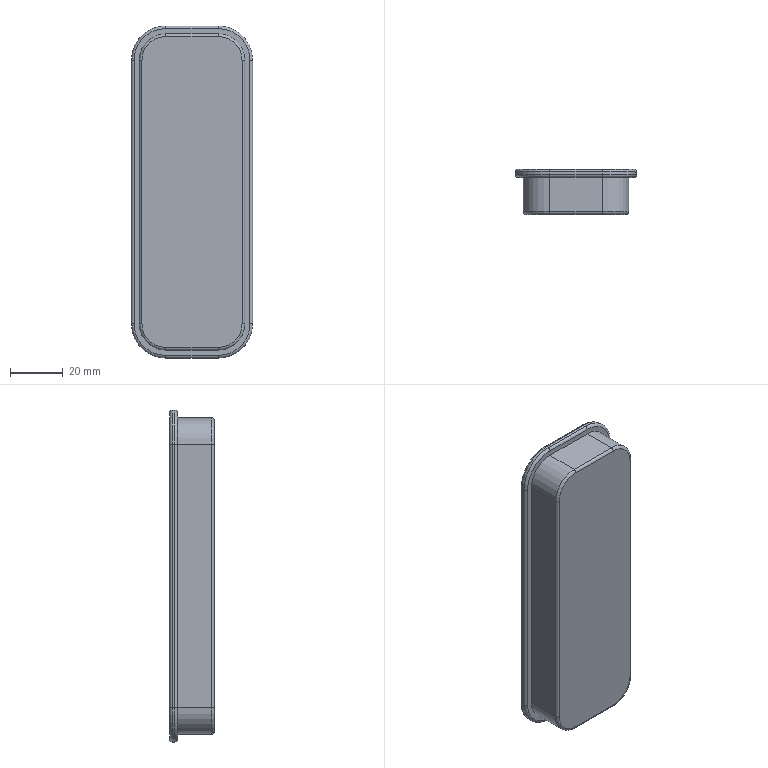Component | SolidWorks | DoorPlate-1_Handle-1 | 1 solid | 91 faces | volume 30524 mm3 | cylinder 43 | torus 28 | plane 20 | commonest cylinder face diameters 2 x27 14 x4 26 x4 6 x4 20 x4